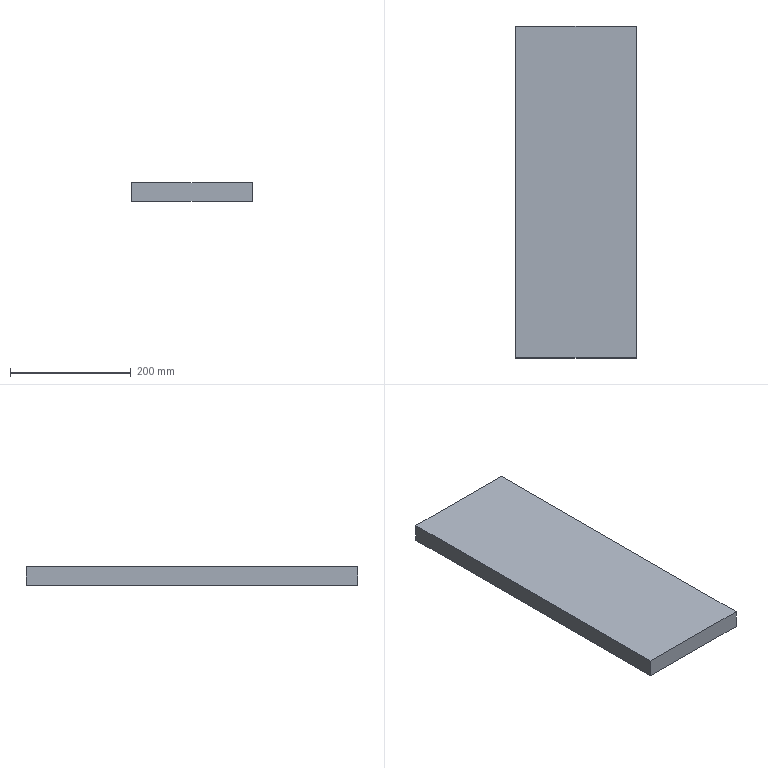Component | SolidWorks | BearingHousing-3_BearingHousingBasePlate-1 | 1 solid | 6 faces | box 200 x 550 x 30 mm | volume 3300000 mm3 | plane 6 | material Plain Carbon Steel
STEP:
#1=CARTESIAN_POINT('',(-250.609,138.257,265.12));
#2=VERTEX_POINT('',#1);
#3=CARTESIAN_POINT('',(-258.483,138.257,265.12));
#4=VERTEX_POINT('',#3);
#5=CARTESIAN_POINT('',(-250.609,138.257,265.12));
#6=DIRECTION('',(-1.,-0.,0.));
#7=VECTOR('',#6,39.37);
#8=LINE('',#5,#7);
#9=EDGE_CURVE('',#2,#4,#8,.T.);
#10=ORIENTED_EDGE('',*,*,#9,.F.);
#11=CARTESIAN_POINT('',(-250.609,138.257,263.939));
#12=VERTEX_POINT('',#11);
#13=CARTESIAN_POINT('',(-250.609,138.257,263.939));
#14=DIRECTION('',(-0.,-0.,1.));
#15=VECTOR('',#14,39.37);
#16=LINE('',#13,#15);
#17=EDGE_CURVE('',#12,#2,#16,.T.);
#18=ORIENTED_EDGE('',*,*,#17,.F.);
#19=CARTESIAN_POINT('',(-258.483,138.257,263.939));
#20=VERTEX_POINT('',#19);
#21=CARTESIAN_POINT('',(-250.609,138.257,263.939));
#22=DIRECTION('',(-1.,-0.,0.));
#23=VECTOR('',#22,39.37);
#24=LINE('',#21,#23);
#25=EDGE_CURVE('',#12,#20,#24,.T.);
#26=ORIENTED_EDGE('',*,*,#25,.T.);
#27=CARTESIAN_POINT('',(-258.483,138.257,263.939));
#28=DIRECTION('',(-0.,-0.,1.));
#29=VECTOR('',#28,39.37);
#30=LINE('',#27,#29);
#31=EDGE_CURVE('',#20,#4,#30,.T.);
#32=ORIENTED_EDGE('',*,*,#31,.T.);
#33=EDGE_LOOP('',(#10,#18,#26,#32));
#34=FACE_OUTER_BOUND('',#33,.T.);
#35=CARTESIAN_POINT('',(-250.609,138.257,263.939));
#36=DIRECTION('',(-0.,1.,0.));
#37=DIRECTION('',(-1.,-0.,0.));
#38=AXIS2_PLACEMENT_3D('',#35,#36,#37);
#39=PLANE('',#38);
#40=ADVANCED_FACE('',(#34),#39,.T.);
#41=CARTESIAN_POINT('',(-250.609,116.604,265.12));
#42=VERTEX_POINT('',#41);
#43=CARTESIAN_POINT('',(-250.609,138.257,265.12));
#44=DIRECTION('',(0.,1.,0.));
#45=VECTOR('',#44,39.37);
#46=LINE('',#43,#45);
#47=EDGE_CURVE('',#42,#2,#46,.T.);
#48=ORIENTED_EDGE('',*,*,#47,.F.);
#49=CARTESIAN_POINT('',(-250.609,116.604,263.939));
#50=VERTEX_POINT('',#49);
#51=CARTESIAN_POINT('',(-250.609,116.604,263.939));
#52=DIRECTION('',(-0.,-0.,1.));
#53=VECTOR('',#52,39.37);
#54=LINE('',#51,#53);
#55=EDGE_CURVE('',#50,#42,#54,.T.);
#56=ORIENTED_EDGE('',*,*,#55,.F.);
#57=CARTESIAN_POINT('',(-250.609,138.257,263.939));
#58=DIRECTION('',(0.,1.,0.));
#59=VECTOR('',#58,39.37);
#60=LINE('',#57,#59);
#61=EDGE_CURVE('',#50,#12,#60,.T.);
#62=ORIENTED_EDGE('',*,*,#61,.T.);
#63=ORIENTED_EDGE('',*,*,#17,.T.);
#64=EDGE_LOOP('',(#48,#56,#62,#63));
#65=FACE_OUTER_BOUND('',#64,.T.);
#66=CARTESIAN_POINT('',(-250.609,138.257,263.939));
#67=DIRECTION('',(1.,-0.,-0.));
#68=DIRECTION('',(0.,1.,0.));
#69=AXIS2_PLACEMENT_3D('',#66,#67,#68);
#70=PLANE('',#69);
#71=ADVANCED_FACE('',(#65),#70,.T.);
#72=CARTESIAN_POINT('',(-258.483,116.604,265.12));
#73=VERTEX_POINT('',#72);
#74=CARTESIAN_POINT('',(-250.609,116.604,265.12));
#75=DIRECTION('',(1.,0.,-0.));
#76=VECTOR('',#75,39.37);
#77=LINE('',#74,#76);
#78=EDGE_CURVE('',#73,#42,#77,.T.);
#79=ORIENTED_EDGE('',*,*,#78,.F.);
#80=CARTESIAN_POINT('',(-258.483,116.604,263.939));
#81=VERTEX_POINT('',#80);
#82=CARTESIAN_POINT('',(-258.483,116.604,263.939));
#83=DIRECTION('',(-0.,-0.,1.));
#84=VECTOR('',#83,39.37);
#85=LINE('',#82,#84);
#86=EDGE_CURVE('',#81,#73,#85,.T.);
#87=ORIENTED_EDGE('',*,*,#86,.F.);
#88=CARTESIAN_POINT('',(-250.609,116.604,263.939));
#89=DIRECTION('',(1.,0.,-0.));
#90=VECTOR('',#89,39.37);
#91=LINE('',#88,#90);
#92=EDGE_CURVE('',#81,#50,#91,.T.);
#93=ORIENTED_EDGE('',*,*,#92,.T.);
#94=ORIENTED_EDGE('',*,*,#55,.T.);
#95=EDGE_LOOP('',(#79,#87,#93,#94));
#96=FACE_OUTER_BOUND('',#95,.T.);
#97=CARTESIAN_POINT('',(-250.609,116.604,263.939));
#98=DIRECTION('',(0.,-1.,-0.));
#99=DIRECTION('',(1.,0.,-0.));
#100=AXIS2_PLACEMENT_3D('',#97,#98,#99);
#101=PLANE('',#100);
#102=ADVANCED_FACE('',(#96),#101,.T.);
#103=CARTESIAN_POINT('',(-258.483,138.257,265.12));
#104=DIRECTION('',(-0.,-1.,-0.));
#105=VECTOR('',#104,39.37);
#106=LINE('',#103,#105);
#107=EDGE_CURVE('',#4,#73,#106,.T.);
#108=ORIENTED_EDGE('',*,*,#107,.F.);
#109=ORIENTED_EDGE('',*,*,#31,.F.);
#110=CARTESIAN_POINT('',(-258.483,138.257,263.939));
#111=DIRECTION('',(-0.,-1.,-0.));
#112=VECTOR('',#111,39.37);
#113=LINE('',#110,#112);
#114=EDGE_CURVE('',#20,#81,#113,.T.);
#115=ORIENTED_EDGE('',*,*,#114,.T.);
#116=ORIENTED_EDGE('',*,*,#86,.T.);
#117=EDGE_LOOP('',(#108,#109,#115,#116));
#118=FACE_OUTER_BOUND('',#117,.T.);
#119=CARTESIAN_POINT('',(-258.483,138.257,263.939));
#120=DIRECTION('',(-1.,0.,0.));
#121=DIRECTION('',(-0.,-1.,-0.));
#122=AXIS2_PLACEMENT_3D('',#119,#120,#121);
#123=PLANE('',#122);
#124=ADVANCED_FACE('',(#118),#123,.T.);
#125=ORIENTED_EDGE('',*,*,#25,.F.);
#126=ORIENTED_EDGE('',*,*,#61,.F.);
#127=ORIENTED_EDGE('',*,*,#92,.F.);
#128=ORIENTED_EDGE('',*,*,#114,.F.);
#129=EDGE_LOOP('',(#125,#126,#127,#128));
#130=FACE_OUTER_BOUND('',#129,.T.);
#131=CARTESIAN_POINT('',(-250.609,138.257,263.939));
#132=DIRECTION('',(0.,-0.,1.));
#133=DIRECTION('',(-1.,-0.,0.));
#134=AXIS2_PLACEMENT_3D('',#131,#132,#133);
#135=PLANE('',#134);
#136=ADVANCED_FACE('',(#130),#135,.F.);
#137=ORIENTED_EDGE('',*,*,#9,.T.);
#138=ORIENTED_EDGE('',*,*,#107,.T.);
#139=ORIENTED_EDGE('',*,*,#78,.T.);
#140=ORIENTED_EDGE('',*,*,#47,.T.);
#141=EDGE_LOOP('',(#137,#138,#139,#140));
#142=FACE_OUTER_BOUND('',#141,.T.);
#143=CARTESIAN_POINT('',(-250.609,138.257,265.12));
#144=DIRECTION('',(0.,-0.,1.));
#145=DIRECTION('',(-1.,-0.,0.));
#146=AXIS2_PLACEMENT_3D('',#143,#144,#145);
#147=PLANE('',#146);
#148=ADVANCED_FACE('',(#142),#147,.T.);
#149=CLOSED_SHELL('',(#40,#71,#102,#124,#136,#148));
#150=MANIFOLD_SOLID_BREP('',#149);
#151=CARTESIAN_POINT('',(0.,0.,0.));
#152=DIRECTION('',(0.,0.,1.));
#153=DIRECTION('',(1.,0.,0.));
#154=AXIS2_PLACEMENT_3D('',#151,#152,#153);
#155=(LENGTH_UNIT()NAMED_UNIT(*)SI_UNIT($,.METRE.));
#156=LENGTH_MEASURE_WITH_UNIT(LENGTH_MEASURE(0.0254),#155);
#157=DIMENSIONAL_EXPONENTS(1.,0.,0.,0.,0.,0.,0.);
#158=(CONVERSION_BASED_UNIT('',#156)LENGTH_UNIT()NAMED_UNIT(#157));
#159=UNCERTAINTY_MEASURE_WITH_UNIT(LENGTH_MEASURE(0.00001),#158,'','');
#160=(NAMED_UNIT(*)PLANE_ANGLE_UNIT()SI_UNIT($,.RADIAN.));
#161=(NAMED_UNIT(*)SI_UNIT($,.STERADIAN.)SOLID_ANGLE_UNIT());
#162=(GEOMETRIC_REPRESENTATION_CONTEXT(3)GLOBAL_UNCERTAINTY_ASSIGNED_CONTEXT((#159))GLOBAL_UNIT_ASSIGNED_CONTEXT((#158,#160,#161))REPRESENTATION_CONTEXT('',''));
#163=ADVANCED_BREP_SHAPE_REPRESENTATION('',(#150,#154),#162);
#164=COLOUR_RGB('',0.7922,0.8196,0.9333);
#165=FILL_AREA_STYLE_COLOUR('',#164);
#166=FILL_AREA_STYLE('',(#165));
#167=SURFACE_STYLE_FILL_AREA(#166);
#168=SURFACE_SIDE_STYLE('',(#167));
#169=SURFACE_STYLE_USAGE(.BOTH.,#168);
#170=PRESENTATION_STYLE_ASSIGNMENT((#169));
#171=STYLED_ITEM('',(#170),#150);
#172=(LENGTH_UNIT()NAMED_UNIT(*)SI_UNIT($,.METRE.));
#173=LENGTH_MEASURE_WITH_UNIT(LENGTH_MEASURE(0.0254),#172);
#174=DIMENSIONAL_EXPONENTS(1.,0.,0.,0.,0.,0.,0.);
#175=(CONVERSION_BASED_UNIT('',#173)LENGTH_UNIT()NAMED_UNIT(#174));
#176=UNCERTAINTY_MEASURE_WITH_UNIT(LENGTH_MEASURE(0.00001),#175,'','');
#177=(NAMED_UNIT(*)PLANE_ANGLE_UNIT()SI_UNIT($,.RADIAN.));
#178=(NAMED_UNIT(*)SI_UNIT($,.STERADIAN.)SOLID_ANGLE_UNIT());
#179=(GEOMETRIC_REPRESENTATION_CONTEXT(3)GLOBAL_UNCERTAINTY_ASSIGNED_CONTEXT((#176))GLOBAL_UNIT_ASSIGNED_CONTEXT((#175,#177,#178))REPRESENTATION_CONTEXT('',''));
#180=MECHANICAL_DESIGN_GEOMETRIC_PRESENTATION_REPRESENTATION('',(#171),#179);
#181=PRESENTATION_LAYER_ASSIGNMENT('','',(#171));